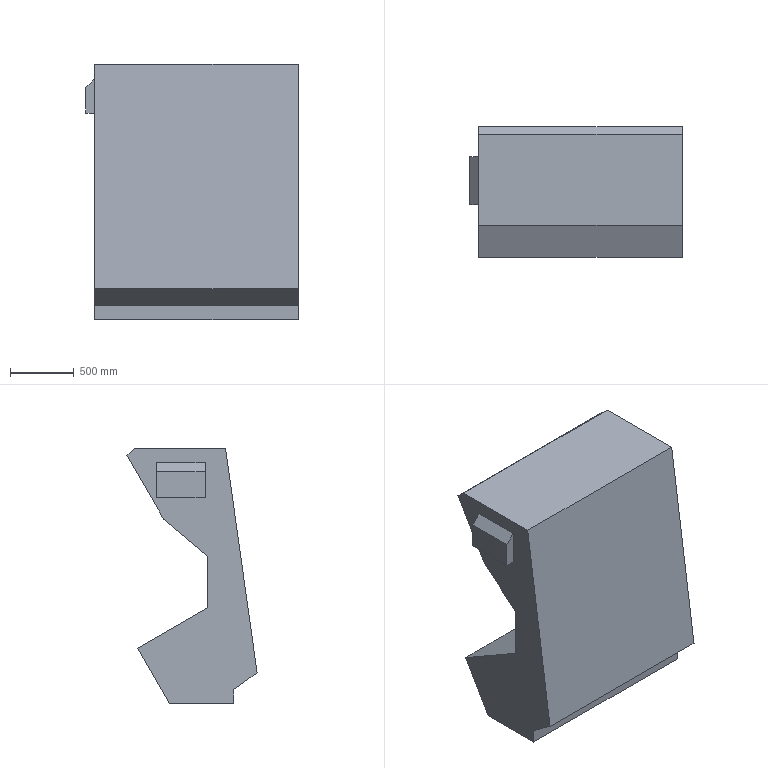Component | NX | SIM15_GEGENSPINDELSEITE | 1 solid | 18 faces | volume 1809789678 mm3 | plane 18